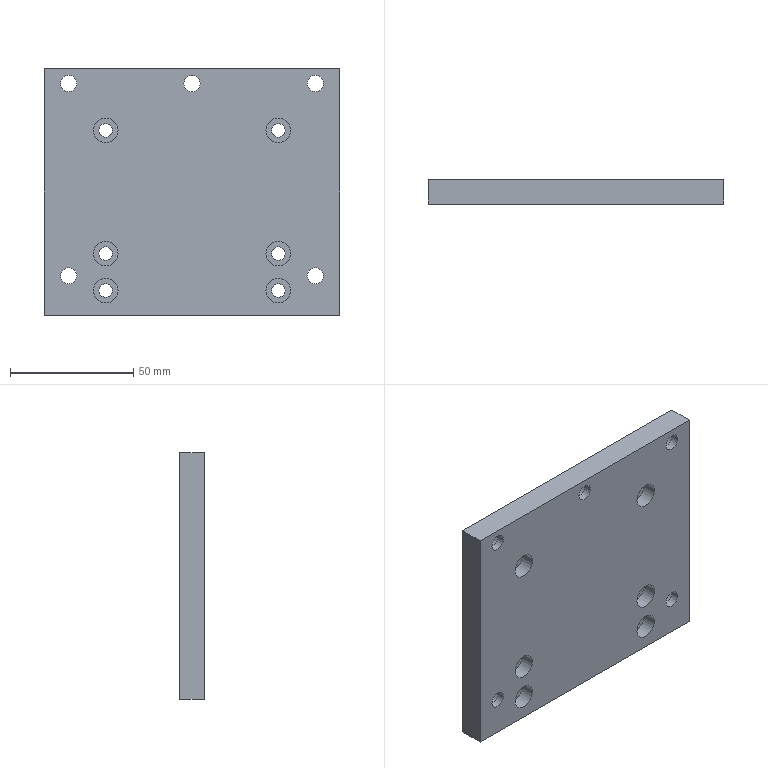Component | SolidWorks | 75-02-11StirringUpperAndLowerMountingPlate-1 | 1 solid | 61 faces | box 120 x 10 x 100 mm | volume 112922 mm3 | cylinder 44 | plane 17 | commonest cylinder face diameters 10 x12 5.5 x12 11 x10 6.6 x10 | material A3 Steel
build123d program:
from build123d import *

# Parameters (mm, degrees)
SKETCH1_W                                          = 120
SKETCH1_H                                          = 100
BOSS_EXTRUDE1_DEPTH                                = 5
HOLE_SIZE_ACCORDING_TO_TYPE_OF_HEXAGON_D           = 6.6
HOLE_SIZE_ACCORDING_TO_TYPE_OF_HEXAGON_CBORE_D     = 11
HOLE_SIZE_ACCORDING_TO_TYPE_OF_HEXAGON_CBORE_DEPTH = 6.8
HOLE_SIZE_ACCORDING_TO_TYPE_OF_HEX_2_D             = 6.6
HOLE_SIZE_ACCORDING_TO_TYPE_OF_HEX_2_CBORE_D       = 11
HOLE_SIZE_ACCORDING_TO_TYPE_OF_HEX_2_CBORE_DEPTH   = 6.8
HOLE_SIZE_ACCORDING_TO_TYPE_OF_HEX_3_D             = 5.5
HOLE_SIZE_ACCORDING_TO_TYPE_OF_HEX_3_CBORE_D       = 10
HOLE_SIZE_ACCORDING_TO_TYPE_OF_HEX_3_CBORE_DEPTH   = 5.7
HOLE_SIZE_ACCORDING_TO_TYPE_OF_HEX_4_D             = 5.5
HOLE_SIZE_ACCORDING_TO_TYPE_OF_HEX_4_CBORE_D       = 10
HOLE_SIZE_ACCORDING_TO_TYPE_OF_HEX_4_CBORE_DEPTH   = 5.7
HOLE_SIZE_ACCORDING_TO_TYPE_OF_HEX_4_O_D           = 5.5
HOLE_SIZE_ACCORDING_TO_TYPE_OF_HEX_4_O_CBORE_D     = 10
HOLE_SIZE_ACCORDING_TO_TYPE_OF_HEX_4_O_CBORE_DEPTH = 5.7


with BuildPart() as part:
    # Sketch1 → Boss-Extrude1 (new, symmetric)
    with BuildSketch(Plane.XY):
        Rectangle(SKETCH1_W, SKETCH1_H)
    extrude(amount=BOSS_EXTRUDE1_DEPTH, both=True)

    # Hole Size _according to_ Type of Hexagon (through all)
    with Locations(Plane(origin=(-50, 44, 5), x_dir=(1, 0, 0), z_dir=(0, 0, 1))):
        with Locations((0, 0), (100, 0), (50, 0)):
            CounterBoreHole(HOLE_SIZE_ACCORDING_TO_TYPE_OF_HEXAGON_D / 2, HOLE_SIZE_ACCORDING_TO_TYPE_OF_HEXAGON_CBORE_D / 2, HOLE_SIZE_ACCORDING_TO_TYPE_OF_HEXAGON_CBORE_DEPTH)

    # Hole Size _according to_ Type of Hex 2 (through all)
    with Locations(Plane(origin=(-50, -34, 5), x_dir=(1, 0, 0), z_dir=(0, 0, 1))):
        with Locations((0, 0), (100, 0)):
            CounterBoreHole(HOLE_SIZE_ACCORDING_TO_TYPE_OF_HEX_2_D / 2, HOLE_SIZE_ACCORDING_TO_TYPE_OF_HEX_2_CBORE_D / 2, HOLE_SIZE_ACCORDING_TO_TYPE_OF_HEX_2_CBORE_DEPTH)

    # Hole Size _according to_ Type of Hex 3 (through all)
    with Locations(Plane(origin=(35, 25, -5), x_dir=(-1, 0, 0), z_dir=(0, 0, -1))):
        with Locations((0, 0), (70, 0), (70, -50), (0, -50)):
            CounterBoreHole(HOLE_SIZE_ACCORDING_TO_TYPE_OF_HEX_3_D / 2, HOLE_SIZE_ACCORDING_TO_TYPE_OF_HEX_3_CBORE_D / 2, HOLE_SIZE_ACCORDING_TO_TYPE_OF_HEX_3_CBORE_DEPTH)

    # Hole Size _according to_ Type of Hex 4 (through all)
    with Locations(Plane(origin=(35, -40, -5), x_dir=(-1, 0, 0), z_dir=(0, 0, -1))):
        with Locations((0, 0), (70, 0)):
            CounterBoreHole(HOLE_SIZE_ACCORDING_TO_TYPE_OF_HEX_4_D / 2, HOLE_SIZE_ACCORDING_TO_TYPE_OF_HEX_4_CBORE_D / 2, HOLE_SIZE_ACCORDING_TO_TYPE_OF_HEX_4_CBORE_DEPTH)

    # Hole Size _according to_ Type of Hex 4 o (through all)
    with Locations(Plane(origin=(75.868, -12.035, 0), x_dir=(-1, 0, 0), z_dir=(0, 0, -1))):
        with Locations((0, 0)):
            CounterBoreHole(HOLE_SIZE_ACCORDING_TO_TYPE_OF_HEX_4_O_D / 2, HOLE_SIZE_ACCORDING_TO_TYPE_OF_HEX_4_O_CBORE_D / 2, HOLE_SIZE_ACCORDING_TO_TYPE_OF_HEX_4_O_CBORE_DEPTH)


solid = part.part

# Placed as in the assembly
solid = solid.moved(Location((-17.8, 121.867, 63.75), (-90, 0, 180)))